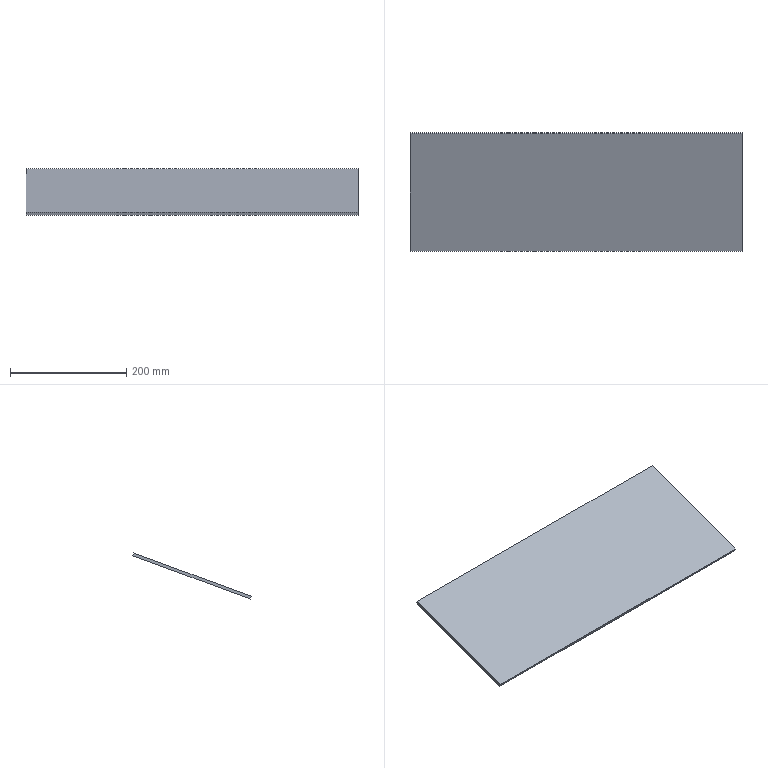Component | SolidWorks | TrashCanDoor-1 | 1 solid | 6 faces | box 570 x 203.44 x 79.12 mm | volume 612750 mm3 | plane 6
build123d program:
from build123d import *

# Parameters (mm, degrees)
SKETCH1_W           = 570
SKETCH1_H           = 215
BOSS_EXTRUDE1_DEPTH = 5


with BuildPart() as part:
    # Sketch1 → Boss-Extrude1 (new body)
    with BuildSketch(Plane.XY):
        Rectangle(SKETCH1_W, SKETCH1_H)
    extrude(amount=BOSS_EXTRUDE1_DEPTH)


solid = part.part

# Placed as in the assembly
solid = solid.moved(Location((25.629, -1454.183, 160.944), (-159.745, 0, 0)))
STEP:
#1=COLOUR_RGB('',0.7922,0.8196,0.9333);
#2=FILL_AREA_STYLE_COLOUR('',#1);
#3=FILL_AREA_STYLE('',(#2));
#4=SURFACE_STYLE_FILL_AREA(#3);
#5=SURFACE_SIDE_STYLE('',(#4));
#6=SURFACE_STYLE_USAGE(.BOTH.,#5);
#7=PRESENTATION_STYLE_ASSIGNMENT((#6));
#8=CARTESIAN_POINT('',(12.23,-53.281,7.802));
#9=VERTEX_POINT('',#8);
#10=CARTESIAN_POINT('',(12.23,-61.222,4.871));
#11=VERTEX_POINT('',#10);
#12=CARTESIAN_POINT('',(12.23,-53.281,7.802));
#13=DIRECTION('',(0.,-0.9382,-0.3462));
#14=VECTOR('',#13,39.37);
#15=LINE('',#12,#14);
#16=EDGE_CURVE('',#9,#11,#15,.T.);
#17=ORIENTED_EDGE('',*,*,#16,.T.);
#18=CARTESIAN_POINT('',(12.23,-61.154,4.686));
#19=VERTEX_POINT('',#18);
#20=CARTESIAN_POINT('',(12.23,-61.154,4.686));
#21=DIRECTION('',(0.,-0.3462,0.9382));
#22=VECTOR('',#21,39.37);
#23=LINE('',#20,#22);
#24=EDGE_CURVE('',#19,#11,#23,.T.);
#25=ORIENTED_EDGE('',*,*,#24,.F.);
#26=CARTESIAN_POINT('',(12.23,-53.213,7.617));
#27=VERTEX_POINT('',#26);
#28=CARTESIAN_POINT('',(12.23,-53.213,7.617));
#29=DIRECTION('',(0.,-0.9382,-0.3462));
#30=VECTOR('',#29,39.37);
#31=LINE('',#28,#30);
#32=EDGE_CURVE('',#27,#19,#31,.T.);
#33=ORIENTED_EDGE('',*,*,#32,.F.);
#34=CARTESIAN_POINT('',(12.23,-53.213,7.617));
#35=DIRECTION('',(0.,-0.3462,0.9382));
#36=VECTOR('',#35,39.37);
#37=LINE('',#34,#36);
#38=EDGE_CURVE('',#27,#9,#37,.T.);
#39=ORIENTED_EDGE('',*,*,#38,.T.);
#40=EDGE_LOOP('',(#17,#25,#33,#39));
#41=FACE_OUTER_BOUND('',#40,.T.);
#42=CARTESIAN_POINT('',(12.23,-53.213,7.617));
#43=DIRECTION('',(-1.,-0.,0.));
#44=DIRECTION('',(-0.,0.3462,-0.9382));
#45=AXIS2_PLACEMENT_3D('',#42,#43,#44);
#46=PLANE('',#45);
#47=ADVANCED_FACE('',(#41),#46,.F.);
#48=CARTESIAN_POINT('',(-10.211,-61.222,4.871));
#49=VERTEX_POINT('',#48);
#50=CARTESIAN_POINT('',(-10.211,-61.222,4.871));
#51=DIRECTION('',(-1.,-0.,0.));
#52=VECTOR('',#51,39.37);
#53=LINE('',#50,#52);
#54=EDGE_CURVE('',#11,#49,#53,.T.);
#55=ORIENTED_EDGE('',*,*,#54,.T.);
#56=CARTESIAN_POINT('',(-10.211,-61.154,4.686));
#57=VERTEX_POINT('',#56);
#58=CARTESIAN_POINT('',(-10.211,-61.154,4.686));
#59=DIRECTION('',(0.,-0.3462,0.9382));
#60=VECTOR('',#59,39.37);
#61=LINE('',#58,#60);
#62=EDGE_CURVE('',#57,#49,#61,.T.);
#63=ORIENTED_EDGE('',*,*,#62,.F.);
#64=CARTESIAN_POINT('',(-10.211,-61.154,4.686));
#65=DIRECTION('',(-1.,-0.,0.));
#66=VECTOR('',#65,39.37);
#67=LINE('',#64,#66);
#68=EDGE_CURVE('',#19,#57,#67,.T.);
#69=ORIENTED_EDGE('',*,*,#68,.F.);
#70=ORIENTED_EDGE('',*,*,#24,.T.);
#71=EDGE_LOOP('',(#55,#63,#69,#70));
#72=FACE_OUTER_BOUND('',#71,.T.);
#73=CARTESIAN_POINT('',(-10.211,-61.154,4.686));
#74=DIRECTION('',(-0.,0.9382,0.3462));
#75=DIRECTION('',(0.,-0.3462,0.9382));
#76=AXIS2_PLACEMENT_3D('',#73,#74,#75);
#77=PLANE('',#76);
#78=ADVANCED_FACE('',(#72),#77,.F.);
#79=CARTESIAN_POINT('',(-10.211,-53.281,7.802));
#80=VERTEX_POINT('',#79);
#81=CARTESIAN_POINT('',(-10.211,-53.281,7.802));
#82=DIRECTION('',(-0.,0.9382,0.3462));
#83=VECTOR('',#82,39.37);
#84=LINE('',#81,#83);
#85=EDGE_CURVE('',#49,#80,#84,.T.);
#86=ORIENTED_EDGE('',*,*,#85,.T.);
#87=CARTESIAN_POINT('',(-10.211,-53.213,7.617));
#88=VERTEX_POINT('',#87);
#89=CARTESIAN_POINT('',(-10.211,-53.213,7.617));
#90=DIRECTION('',(0.,-0.3462,0.9382));
#91=VECTOR('',#90,39.37);
#92=LINE('',#89,#91);
#93=EDGE_CURVE('',#88,#80,#92,.T.);
#94=ORIENTED_EDGE('',*,*,#93,.F.);
#95=CARTESIAN_POINT('',(-10.211,-53.213,7.617));
#96=DIRECTION('',(-0.,0.9382,0.3462));
#97=VECTOR('',#96,39.37);
#98=LINE('',#95,#97);
#99=EDGE_CURVE('',#57,#88,#98,.T.);
#100=ORIENTED_EDGE('',*,*,#99,.F.);
#101=ORIENTED_EDGE('',*,*,#62,.T.);
#102=EDGE_LOOP('',(#86,#94,#100,#101));
#103=FACE_OUTER_BOUND('',#102,.T.);
#104=CARTESIAN_POINT('',(-10.211,-53.213,7.617));
#105=DIRECTION('',(1.,0.,-0.));
#106=DIRECTION('',(0.,-0.3462,0.9382));
#107=AXIS2_PLACEMENT_3D('',#104,#105,#106);
#108=PLANE('',#107);
#109=ADVANCED_FACE('',(#103),#108,.F.);
#110=CARTESIAN_POINT('',(-10.211,-53.281,7.802));
#111=DIRECTION('',(1.,0.,-0.));
#112=VECTOR('',#111,39.37);
#113=LINE('',#110,#112);
#114=EDGE_CURVE('',#80,#9,#113,.T.);
#115=ORIENTED_EDGE('',*,*,#114,.T.);
#116=ORIENTED_EDGE('',*,*,#38,.F.);
#117=CARTESIAN_POINT('',(-10.211,-53.213,7.617));
#118=DIRECTION('',(1.,0.,-0.));
#119=VECTOR('',#118,39.37);
#120=LINE('',#117,#119);
#121=EDGE_CURVE('',#88,#27,#120,.T.);
#122=ORIENTED_EDGE('',*,*,#121,.F.);
#123=ORIENTED_EDGE('',*,*,#93,.T.);
#124=EDGE_LOOP('',(#115,#116,#122,#123));
#125=FACE_OUTER_BOUND('',#124,.T.);
#126=CARTESIAN_POINT('',(-10.211,-53.213,7.617));
#127=DIRECTION('',(0.,-0.9382,-0.3462));
#128=DIRECTION('',(-0.,0.3462,-0.9382));
#129=AXIS2_PLACEMENT_3D('',#126,#127,#128);
#130=PLANE('',#129);
#131=ADVANCED_FACE('',(#125),#130,.F.);
#132=ORIENTED_EDGE('',*,*,#32,.T.);
#133=ORIENTED_EDGE('',*,*,#68,.T.);
#134=ORIENTED_EDGE('',*,*,#99,.T.);
#135=ORIENTED_EDGE('',*,*,#121,.T.);
#136=EDGE_LOOP('',(#132,#133,#134,#135));
#137=FACE_OUTER_BOUND('',#136,.T.);
#138=CARTESIAN_POINT('',(1.009,-57.183,6.152));
#139=DIRECTION('',(0.,-0.3462,0.9382));
#140=DIRECTION('',(-1.,-0.,0.));
#141=AXIS2_PLACEMENT_3D('',#138,#139,#140);
#142=PLANE('',#141);
#143=ADVANCED_FACE('',(#137),#142,.F.);
#144=ORIENTED_EDGE('',*,*,#16,.F.);
#145=ORIENTED_EDGE('',*,*,#114,.F.);
#146=ORIENTED_EDGE('',*,*,#85,.F.);
#147=ORIENTED_EDGE('',*,*,#54,.F.);
#148=EDGE_LOOP('',(#144,#145,#146,#147));
#149=FACE_OUTER_BOUND('',#148,.T.);
#150=CARTESIAN_POINT('',(1.009,-57.251,6.336));
#151=DIRECTION('',(0.,-0.3462,0.9382));
#152=DIRECTION('',(-1.,-0.,0.));
#153=AXIS2_PLACEMENT_3D('',#150,#151,#152);
#154=PLANE('',#153);
#155=ADVANCED_FACE('',(#149),#154,.T.);
#156=CLOSED_SHELL('',(#47,#78,#109,#131,#143,#155));
#157=MANIFOLD_SOLID_BREP('',#156);
#158=STYLED_ITEM('',(#7),#157);
#159=PRESENTATION_LAYER_ASSIGNMENT('','',(#158));
#160=CARTESIAN_POINT('',(0.,0.,0.));
#161=DIRECTION('',(0.,0.,1.));
#162=DIRECTION('',(1.,0.,0.));
#163=AXIS2_PLACEMENT_3D('',#160,#161,#162);
#164=(LENGTH_UNIT()NAMED_UNIT(*)SI_UNIT($,.METRE.));
#165=LENGTH_MEASURE_WITH_UNIT(LENGTH_MEASURE(0.0254),#164);
#166=DIMENSIONAL_EXPONENTS(1.,0.,0.,0.,0.,0.,0.);
#167=(CONVERSION_BASED_UNIT('',#165)LENGTH_UNIT()NAMED_UNIT(#166));
#168=UNCERTAINTY_MEASURE_WITH_UNIT(LENGTH_MEASURE(0.00001),#167,'','');
#169=(NAMED_UNIT(*)PLANE_ANGLE_UNIT()SI_UNIT($,.RADIAN.));
#170=(NAMED_UNIT(*)SI_UNIT($,.STERADIAN.)SOLID_ANGLE_UNIT());
#171=(GEOMETRIC_REPRESENTATION_CONTEXT(3)GLOBAL_UNCERTAINTY_ASSIGNED_CONTEXT((#168))GLOBAL_UNIT_ASSIGNED_CONTEXT((#167,#169,#170))REPRESENTATION_CONTEXT('',''));
#172=ADVANCED_BREP_SHAPE_REPRESENTATION('',(#157,#163),#171);
#173=(LENGTH_UNIT()NAMED_UNIT(*)SI_UNIT($,.METRE.));
#174=LENGTH_MEASURE_WITH_UNIT(LENGTH_MEASURE(0.0254),#173);
#175=DIMENSIONAL_EXPONENTS(1.,0.,0.,0.,0.,0.,0.);
#176=(CONVERSION_BASED_UNIT('',#174)LENGTH_UNIT()NAMED_UNIT(#175));
#177=UNCERTAINTY_MEASURE_WITH_UNIT(LENGTH_MEASURE(0.00001),#176,'','');
#178=(NAMED_UNIT(*)PLANE_ANGLE_UNIT()SI_UNIT($,.RADIAN.));
#179=(NAMED_UNIT(*)SI_UNIT($,.STERADIAN.)SOLID_ANGLE_UNIT());
#180=(GEOMETRIC_REPRESENTATION_CONTEXT(3)GLOBAL_UNCERTAINTY_ASSIGNED_CONTEXT((#177))GLOBAL_UNIT_ASSIGNED_CONTEXT((#176,#178,#179))REPRESENTATION_CONTEXT('',''));
#181=MECHANICAL_DESIGN_GEOMETRIC_PRESENTATION_REPRESENTATION('',(#158),#180);